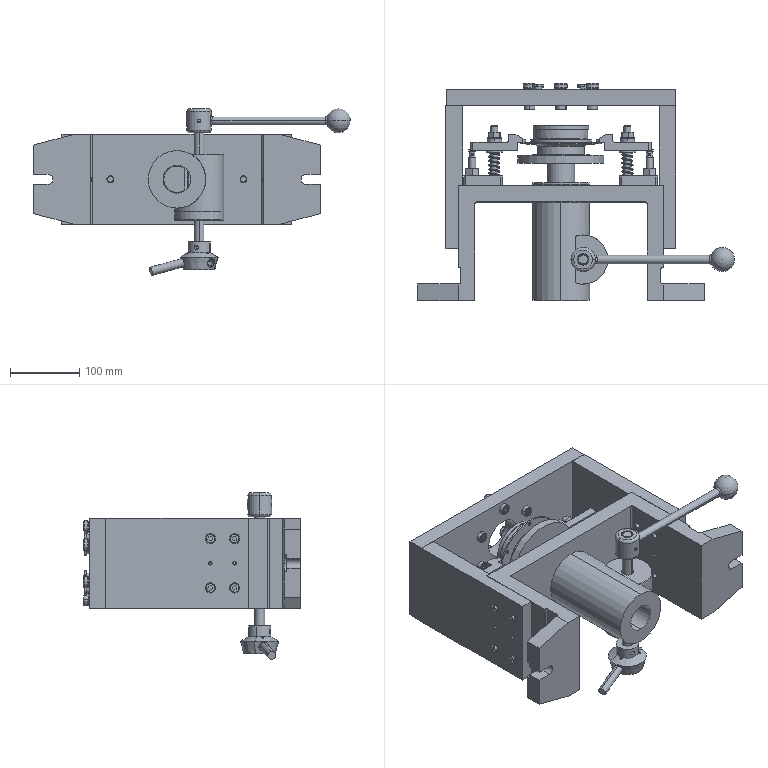Assembly | SolidWorks | mm | 72 component files | 73 solids | 1770 faces | box 457.51 x 313.05 x 240.63 mm | volume 5623344 mm3 | plane 629 | cylinder 586 | cone 407 | torus 132 | sphere 10 | spline 6 | commonest cylinder face diameters 15 x82 10 x68 5 x60 8 x58 6 x28 9 x24 9.5 x24 13 x24
Bill of materials:
CylindricalHelicalCompressionSpring | 2 |  | Helical coil of round wire with constant diameter and roughly uniform pitch, about six turns, with open cut ends.
CylindricalPin-UnhardenedSteelAndAusteniticStainlessSteel5_20 | 4 |  | Short solid cylindrical pin with a small chamfer at both ends. Its length is about four times its diameter.
CylindricalPin-UnhardenedSteelAndAusteniticStainlessSteel5_35 | 3 |  | Slender solid cylindrical pin with small chamfers at both ends. Its length is about seven times its diameter.
DrillJigBody | 1 |  | U-shaped channel bracket. Outward flanges at its base each have an open-ended slot. The side walls have small holes. A cylindrical boss with an axial through bore and a small radial cross hole sits inside the channel.
DrillTemplate | 1 |  | Flat rectangular plate with a large central through hole. Six smaller holes are spaced evenly around the central hole, and there are further holes near both short edges.
GB_T_70.1-2008[SocketHeadCapScrew_M4_20] | 3 |  | Solid of revolution with a short, larger-diameter cylindrical head and a smooth, plain cylindrical shank; the free end of the shank is chamfered. Looks like a headed screw blank or headed pin.
GB_T_70.1-2008[SocketHeadCapScrew_M8_30] | 12 |  | Socket-head-style fastener shape: a cylindrical head with a hexagonal recess in its end face, a smooth cylindrical shank, and a chamfered shank tip. Thread geometry is not modeled.
GB_T15389-1994ScrewM10_100 | 2 |  | Slender solid cylindrical pin. One end has a longer taper or chamfer than the other, which has a small chamfer.
GB_T6170-2000Type1HexNutA-gradeAndB-gradeM10 | 2 |  | Hexagonal nut-like body with a central round through bore. The axial length is short compared with the across-flats width, and the corners are chamfered.
GB_T6170-2015[Type1HexNutM12] | 2 |  | Hexagonal nut-like body with a central round through bore. Both ends have curved corner chamfers, and it is taller relative to its width than unnamed part.
GB_T95-2002[FlatWasherC-grade12] | 2 |  | Flat annular washer-like ring with a plain round central hole.
Handle | 1 |  | Lever or handle with a cylindrical hub at one end, a slender straight rod, and a spherical knob at the other end. The hub has an axial through bore and a small radial cross hole.
HandleRod10InMulti-HandleNut | 1 | Nickel | Solid stepped cylindrical shaft or pin: a long larger-diameter section with a shorter reduced-diameter section at one end.
Handwheel | 1 |  | Shaft carrying a toothed section like a spur gear next to a barrel-shaped (convex) section. There is a small cross hole near one end of the shaft.
JB_T8010.10-1999ElbowClampPlateTypeA12 | 2 | Nickel | Elongated prismatic block with chamfered corners in plan, a central oblong (stadium) through-slot, and a stepped, hook-like end profile in side view.
JB_T8013.1-1999LocatingBushingA18 | 6 | Nickel | Plain hollow cylindrical tube/sleeve with small chamfers at both ends.
Adjusting Support M16 | 2 | Nickel | Long cylindrical pin. At one end is a domed head with a short collar, then a reduced-diameter neck with a transverse through-hole, then a long main body ending in a chamfered tip.
JB_T8045.3-1999QuickChangeDrillBushing10_5_30 | 6 | Nickel | Headed cylindrical pin resembling a cap-screw form: chamfered cylindrical head, short reduced collar/undercut beneath it, plain shank with chamfered tip, and an axial bore; the head appears partially cut away.
JB_T8045.5-1999DrillBushingScrewM6 | 6 | Nickel | Stepped turned pin with a large disc-shaped head, an intermediate cylindrical step, a neck groove, and a chamfered small-diameter pin end; a small notch is cut into the head rim.
LocatingAxis | 1 |  | Pin with a thin large-diameter flat disc head and a cylindrical shank having a flat along part of its side and thread-like serrations near the free end.
LocatingPinAxis | 1 |  | Large chamfered disc with a small stepped hub on one face, comprising a thin flange ring and a short chamfered cylindrical stub.
Nut15InMulti-HandleNut | 1 | Nickel | Turned hub with a cylindrical boss on top of a frustoconical/flared base, a central through bore, radial holes in boss and base, and three axial holes in the base.
PressurePlateFixingSeat | 2 |  | Rectangular block with chamfered corners in plan and two round through holes along its long axis.
SealingCover | 1 |  | Flat circular flange/disc with a central through hole, an annular recess or counterbore on one face, and three small through holes evenly spaced near the perimeter.
SphericalWasherA21 | 2 | Nickel | Dished/conical washer with a convex curved face, flat opposite face, thin cylindrical outer rim, and central hole.
SphericalWasherB21 | 2 | Nickel | Plain flat annular ring/washer with rectangular cross-section.
SupportPlate | 2 |  | Rectangular plate with a thickness step across its width and a pattern of six through holes in two columns of three (four larger, two smaller in the middle row).
TurbineBearingHousing | 1 |  | Thin-walled, axisymmetric, open-ended tubular spigot with a thin flat annular flange. The flange has six evenly spaced through-holes on a bolt circle. On one side of the flange the sleeve steps out to a short collar of larger diameter, then into a main cylindrical section with a slightly raised lip at its far end. On the other side a short tapered shoulder leads to a plain cylindrical sleeve. There is a small oblong slot in the wall near the collar.
Mates:
1. coordinate | DrillJigBody-1 sketch point at (0, 0, 0) dir (1, 0, 0) | assembly sketch point at (0, 0, 0) dir (1, 0, 0)
2. concentric | DrillJigBody-1 face at (-147.862, 95, 35.5) dir (-1, 0, 0) r 4 | SupportPlate-1 face at (-165.862, 95, 35.5) dir (-1, 0, 0) r 7.5
3. concentric | DrillJigBody-1 face at (-147.862, 95, -35.5) dir (-1, 0, 0) r 4 | SupportPlate-1 face at (-165.862, 95, -35.5) dir (-1, 0, 0) r 4.5
4. coincident | DrillJigBody-1 face at (-147.862, 47.316, 65) dir (-1, 0, 0) | SupportPlate-1 face at (-147.862, 75, -99) dir (1, 0, 0)
5. concentric | DrillJigBody-1 face at (0, -23.394, 0) dir (0, 1, 0) r 20 | assembly face at (0, 30.606, 0) dir (0, 1, 0) r 23.5
6. parallel | assembly plane at (0, 197.606, 0) dir (-1, 0, 0) | assembly plane at (0, 0, 0) dir (1, 0, 0)
7. distance | assembly face at (0, 185.606, 0) dir (0, -1, 0) | DrillJigBody-1 face at (0, 169.606, 0) dir (0, 1, 0)
8. concentric | TurbineBearingHousing-1 face at (0, 209.806, 0) dir (0, -1, 0) r 33.75 | DrillJigBody-1 face at (0, -0.05241, 0) dir (0, 1, 0) r 41.5
9. distance | TurbineBearingHousing-1 face at (-57.998, 227.606, -0.4799) dir (0, 1, 0) | DrillJigBody-1 face at (-147.862, 165.606, 65) dir (0, 1, 0)
10. distance | assembly face at (29.76, 42.6, 59) dir (0, 0, 1) | DrillJigBody-1 face at (32, 58.948, 47) dir (0, 0, 1)
11. concentric | DrillJigBody-1 face at (32, 58.948, 81.865) dir (0, 0, 1) r 17.918 | assembly face at (32, 58.948, 112) dir (0, 0, -1) r 7.5
12. concentric | assembly face at (32, 58.948, 112) dir (0, 0, -1) r 7.5 | assembly face at (32, 58.948, 59) dir (0, 0, 1) r 7.5
13. concentric | DrillJigBody-1 face at (32, 29.448, 47) dir (0, 0, 1) r 1.65 | assembly face at (32, 29.448, 59) dir (0, 0, 1) r 2.25
14. coincident | DrillJigBody-1 face at (32, 58.948, 47) dir (0, 0, 1) | assembly face at (32, 58.948, 47) dir (0, 0, -1)
15. concentric | assembly face at (32, 58.948, 112) dir (0, 0, -1) r 7.5 | assembly face at (32, 58.948, 130.416) dir (0, 0, 1) r 9
16. distance | assembly face at (32, 58.948, 112) dir (0, 0, 1) | assembly face at (32, 58.948, 130.416) dir (0, 0, 1)
17. concentric | assembly face at (55.39, 68.739, 120.416) dir (0.891, 0.373, 0.2588) r 5 | assembly face at (53.608, 67.993, 119.898) dir (-0.891, -0.373, -0.2588) r 5
18. coincident | assembly face at (54.382, 64.065, 122.893) dir (0.891, 0.373, 0.2588) | assembly face at (53.608, 67.993, 119.898) dir (-0.891, -0.373, -0.2588)
19. concentric | SupportPlate-1 face at (-153.5, 281, 27.5) dir (0, 1, 0) r 4 | DrillTemplate-1 face at (-153.5, 305, 27.5) dir (0, 1, 0) r 7.5
20. concentric | SupportPlate-1 face at (-153.5, 281, -27.5) dir (0, 1, 0) r 4 | DrillTemplate-1 face at (-153.5, 305, -27.5) dir (0, 1, 0) r 7.5
21. coincident | SupportPlate-1 face at (-141.862, 281, -65) dir (0, 1, 0) | DrillTemplate-1 face at (0, 281, 0) dir (0, -1, 0)
22. concentric | DrillTemplate-1 face at (0, 305, 52.5) dir (0, 1, 0) r 7.5 | JB_T8013.1-1999LocatingBushingA18-1 face at (0, 275, 52.5) dir (0, 1, 0) r 7.5
23. coincident | DrillTemplate-1 face at (0, 305, 0) dir (0, 1, 0) | JB_T8013.1-1999LocatingBushingA18-1 face at (0, 305, 52.5) dir (0, 1, 0)
24. concentric | JB_T8013.1-1999LocatingBushingA18-1 face at (0, 275, 52.5) dir (0, 1, 0) r 5 | JB_T8045.3-1999QuickChangeDrillBushing10_5_30-1 face at (0, 415.352, 52.5) dir (0, 1, 0) r 5
25. coincident | JB_T8013.1-1999LocatingBushingA18-1 face at (0, 305, 52.5) dir (0, 1, 0) | JB_T8045.3-1999QuickChangeDrillBushing10_5_30-1 face at (0, 305, 45) dir (0, -1, 0)
26. parallel | DrillTemplate-1 face at (-165.5, 281, 65) dir (0, 0, 1) | JB_T8045.3-1999QuickChangeDrillBushing10_5_30-1 face at (68.423, 408, 47) dir (0, 0, -1)
27. concentric | DrillTemplate-1 face at (0, 305, 37.5) dir (0, 1, 0) r 3 | JB_T8045.5-1999DrillBushingScrewM6-1 face at (0, 294, 37.5) dir (0, 1, 0) r 3
28. coincident | JB_T8045.3-1999QuickChangeDrillBushing10_5_30-1 face at (68.423, 308, 47) dir (0, 1, 0) | JB_T8045.5-1999DrillBushingScrewM6-1 face at (0, 308, 37.5) dir (0, -1, 0)
29. angle | JB_T8045.5-1999DrillBushingScrewM6-1 face at (17.932, 310, 56.492) dir (0.7071, 0, -0.7071) | JB_T8045.3-1999QuickChangeDrillBushing10_5_30-1 face at (68.423, 408, 47) dir (0, 0, -1)
30. parallel | TurbineBearingHousing-1 face at (-0.4344, 227.606, 52.498) dir (0, 1, 0) r 2.75 | JB_T8045.3-1999QuickChangeDrillBushing10_5_30-1 face at (0, 415.352, 52.5) dir (0, 1, 0) r 2.5
31. concentric | DrillJigBody-1 face at (96, 165.606, 0) dir (0, 1, 0) r 5 | JB_T8010.10-1999ElbowClampPlateTypeA12-1 face at (96, 223.606, 0) dir (0, -1, 0) r 7.5
32. coincident | TurbineBearingHousing-1 face at (-57.998, 227.606, -0.4799) dir (0, 1, 0) | JB_T8010.10-1999ElbowClampPlateTypeA12-1 face at (51, 227.606, 16) dir (0, -1, 0)
33. parallel | SupportPlate-2 face at (141.862, 75, 65) dir (0, 0, 1) | JB_T8010.10-1999ElbowClampPlateTypeA12-1 face at (51, 223.606, 16) dir (0, 0, 1)
34. concentric | DrillJigBody-1 face at (128, 165.606, 0) dir (0, 1, 0) r 5 | JB_T8026.4-1999AdjustingSupportM10_40-1 face at (128, 262.155, 0) dir (0, 1, 0) r 5
35. tangent | JB_T8010.10-1999ElbowClampPlateTypeA12-1 face at (51, 218.606, 0) dir (0, -1, 0) | JB_T8026.4-1999AdjustingSupportM10_40-1 face at (128, 208.606, 0) dir (1, 0, 0) r 10
36. concentric | DrillJigBody-1 face at (96, 165.606, 0) dir (0, 1, 0) r 5 | GB_T15389-1994ScrewM10_100-1 face at (96, 171.901, 0) dir (0, 1, 0) r 5
37. distance | GB_T15389-1994ScrewM10_100-1 face at (96, 251.901, 0) dir (0, 1, 0) | GB_T6170-2000Type1HexNutA-gradeAndB-gradeM10-3 face at (87.661, 242.901, -3.066) dir (0, 1, 0)
38. concentric | GB_T15389-1994ScrewM10_100-1 face at (96, 171.901, 0) dir (0, 1, 0) r 5 | assembly face at (96, 174.006, 0) dir (0, -1, 0) r 5
39. coincident | DrillJigBody-1 face at (-147.862, 165.606, 65) dir (0, 1, 0) | assembly face at (103.712, 165.606, -4.412) dir (0, -1, 0)
40. concentric | JB_T8026.4-1999AdjustingSupportM10_40-1 face at (128, 262.155, 0) dir (0, 1, 0) r 5 | assembly face at (128, 165.606, 0) dir (0, 1, 0) r 5
41. coincident | DrillJigBody-1 face at (-147.862, 165.606, 65) dir (0, 1, 0) | assembly face at (123.957, 165.606, -7.912) dir (0, -1, 0)
42. concentric | GB_T15389-1994ScrewM10_100-1 face at (96, 171.901, 0) dir (0, 1, 0) r 5 | SphericalWasherB21-1 face at (96, 238.624, 0) dir (0, 1, 0) r 5.75
43. coincident | JB_T8010.10-1999ElbowClampPlateTypeA12-1 face at (131, 228.606, -16) dir (0, 1, 0) | SphericalWasherB21-1 face at (101.75, 228.606, 0) dir (0, -1, 0)
44. concentric | GB_T15389-1994ScrewM10_100-1 face at (96, 171.901, 0) dir (0, 1, 0) r 5 | SphericalWasherA21-1 face at (96, 230.466, 0) dir (0, -1, 0) r 5.25
45. tangent | SphericalWasherA21-1 face at (96, 244.553, 0) dir (1, 0, 0) r 15 | SphericalWasherB21-1 face at (96, 233.006, 0) dir (0, -1, 0) r 1047.198
46. concentric | GB_T15389-1994ScrewM10_100-1 face at (96, 171.901, 0) dir (0, 1, 0) r 5 | GB_T6170-2000Type1HexNutA-gradeAndB-gradeM10-3 face at (96, 234.501, 0) dir (0, 1, 0) r 5
47. coincident | SphericalWasherA21-1 face at (97.393, 234.501, -5.062) dir (0, 1, 0) | GB_T6170-2000Type1HexNutA-gradeAndB-gradeM10-3 face at (87.661, 234.501, -3.066) dir (0, -1, 0)
48. concentric | assembly face at (32, 58.948, -20) dir (0, 0, -1) r 7.5 | Handle-1 face at (32, 58.948, 102) dir (0, 0, -1) r 17.5
49. coincident | Handle-1 face at (32, 58.948, 102) dir (0, 0, 1) | Handwheel-2 face at (32, 58.948, 102) dir (0, 0, 1)
50. parallel | DrillTemplate-1 face at (0, 305, 0) dir (0, 1, 0) | Handle-1 plane at (32, 58.948, 84.5) dir (0, -1, 0)
51. concentric | Nut15InMulti-HandleNut-3 face at (32, 58.948, -130.416) dir (0, 0, -1) r 9 | Handwheel-2 face at (32, 58.948, -112) dir (0, 0, 1) r 7.5
52. concentric | SealingCover-2 face at (32, 58.948, -59) dir (0, 0, -1) r 7.5 | Handwheel-2 face at (32, 58.948, -112) dir (0, 0, 1) r 7.5
53. distance | Handwheel-2 face at (32, 58.948, -112) dir (0, 0, -1) | Nut15InMulti-HandleNut-3 face at (32, 58.948, -130.416) dir (0, 0, -1)
54. coincident | HandleRod10InMulti-HandleNut-2 face at (9.315, 53.107, -119.898) dir (0.9354, 0.2408, 0.2588) | Nut15InMulti-HandleNut-3 face at (11.071, 49.509, -122.893) dir (-0.9354, -0.2408, -0.2588)
55. concentric | HandleRod10InMulti-HandleNut-2 face at (9.315, 53.107, -119.898) dir (0.9354, 0.2408, 0.2588) r 5 | Nut15InMulti-HandleNut-3 face at (7.444, 52.625, -120.416) dir (-0.9354, -0.2408, -0.2588) r 5
56. concentric | DrillJigBody-1 face at (32, 58.948, 36) dir (0, 0, -1) r 35.5 | Handwheel-2 face at (32, 58.948, -112) dir (0, 0, 1) r 7.5
57. coincident | DrillJigBody-1 face at (32, 58.948, -47) dir (0, 0, -1) | SealingCover-2 face at (32, 58.948, -47) dir (0, 0, 1)
58. concentric | DrillJigBody-1 face at (32, 29.448, -47) dir (0, 0, -1) r 2 | SealingCover-2 face at (32, 29.448, -59) dir (0, 0, -1) r 4
59. distance | Handwheel-2 face at (32, 58.948, 102) dir (0, 0, 1) | DrillJigBody-1 face at (121.838, 139.582, 65) dir (0, 0, 1)
60. concentric | Handle-1 face at (32, 58.948, 102) dir (0, 0, -1) r 17.5 | Handwheel-2 face at (32, 58.948, 20) dir (0, 0, 1) r 7.5
61. concentric | Handle-1 face at (32, 76.448, 84.5) dir (0, -1, 0) r 2.5 | Handwheel-2 face at (32, 39.338, 84.5) dir (0, 1, 0) r 2.5
62. concentric | Handle-1 face at (32, 76.448, 84.5) dir (0, -1, 0) r 2.5 | CylindricalPin-UnhardenedSteelAndAusteniticStainlessSteel5_35-1 face at (32, 41.448, 84.5) dir (0, 1, 0) r 2.5
63. tangent | Handle-1 face at (32, 58.948, 102) dir (0, 0, -1) r 17.5 | CylindricalPin-UnhardenedSteelAndAusteniticStainlessSteel5_35-1 face at (32, 76.448, 84.5) dir (0, 1, 0)
64. concentric | SupportPlate-2 face at (165.862, 130, 0) dir (1, 0, 0) r 2.5 | CylindricalPin-UnhardenedSteelAndAusteniticStainlessSteel5_20-1 face at (159.862, 130, 0) dir (-1, 0, 0) r 2.5
65. distance | CylindricalPin-UnhardenedSteelAndAusteniticStainlessSteel5_20-1 face at (159.862, 130, 0) dir (1, 0, 0) | SupportPlate-2 face at (165.862, 75, 0) dir (1, 0, 0)
66. concentric | SupportPlate-2 face at (165.862, 95, 0) dir (1, 0, 0) r 2.5 | CylindricalPin-UnhardenedSteelAndAusteniticStainlessSteel5_20-2 face at (159.862, 95, 0) dir (-1, 0, 0) r 2.5
67. distance | CylindricalPin-UnhardenedSteelAndAusteniticStainlessSteel5_20-2 face at (159.862, 95, 0) dir (1, 0, 0) | SupportPlate-2 face at (165.862, 75, 0) dir (1, 0, 0)
68. coincident | SupportPlate-2 face at (156.862, 130, 31) dir (1, 0, 0) | GB_T_70.1-2008[SocketHeadCapScrew_M8_30]-1 face at (156.862, 127.518, 41.507) dir (-1, 0, 0)
69. concentric | SupportPlate-2 face at (165.862, 130, 35.5) dir (1, 0, 0) r 7.5 | GB_T_70.1-2008[SocketHeadCapScrew_M8_30]-1 face at (164.862, 130, 35.5) dir (-1, 0, 0) r 4
70. coincident | DrillJigBody-1 face at (-147.862, 165.606, 65) dir (0, 1, 0) | PressurePlateFixingSeat-1 face at (112, 165.606, 0) dir (0, -1, 0)
71. concentric | GB_T15389-1994ScrewM10_100-1 face at (96, 171.901, 0) dir (0, 1, 0) r 5 | PressurePlateFixingSeat-1 face at (96, 179.606, 0) dir (0, 1, 0) r 5.1
72. parallel | SupportPlate-2 face at (141.862, 75, 0) dir (-1, 0, 0) | PressurePlateFixingSeat-1 face at (84, 179.606, 15) dir (-1, 0, 0)
73. concentric | JB_T8026.4-1999AdjustingSupportM10_40-1 face at (128, 262.155, 0) dir (0, 1, 0) r 5 | GB_T6170-2015[Type1HexNutM12]-1 face at (128, 190.406, 0) dir (0, -1, 0) r 5.053
74. coincident | PressurePlateFixingSeat-1 face at (112, 179.606, 0) dir (0, 1, 0) | GB_T6170-2015[Type1HexNutM12]-1 face at (128, 179.606, 10.392) dir (0, -1, 0)
75. concentric | GB_T15389-1994ScrewM10_100-1 face at (96, 171.901, 0) dir (0, 1, 0) r 5 | GB_T95-2002[FlatWasherC-grade12]-1 face at (96, 205.461, 0) dir (0, -1, 0) r 12
76. coincident | JB_T8010.10-1999ElbowClampPlateTypeA12-1 face at (51, 216.606, 0) dir (0, -1, 0) | GB_T95-2002[FlatWasherC-grade12]-1 face at (89.25, 216.606, 0) dir (0, 1, 0)
77. concentric | GB_T15389-1994ScrewM10_100-1 face at (96, 171.901, 0) dir (0, 1, 0) r 5 | CylindricalHelicalCompressionSpring-1 axis at (96, 216.356, 0) dir (0, -1, 0)
78. coincident | GB_T95-2002[FlatWasherC-grade12]-1 face at (89.25, 214.106, 0) dir (0, -1, 0) | CylindricalHelicalCompressionSpring-1 face at (86.712, 214.106, -8) dir (0, 1, 0)
79. concentric | DrillTemplate-1 face at (-153.5, 305, -48) dir (0, 1, 0) r 2.5 | CylindricalPin-UnhardenedSteelAndAusteniticStainlessSteel5_35-2 face at (-153.5, 305, -48) dir (0, -1, 0) r 2.5
80. coincident | DrillTemplate-1 face at (0, 305, 0) dir (0, 1, 0) | CylindricalPin-UnhardenedSteelAndAusteniticStainlessSteel5_35-2 face at (-153.5, 305, -48) dir (0, 1, 0)
81. concentric | DrillTemplate-1 face at (-153.5, 305, 48) dir (0, 1, 0) r 2.5 | CylindricalPin-UnhardenedSteelAndAusteniticStainlessSteel5_35-3 face at (-153.5, 305, 48) dir (0, -1, 0) r 2.5
82. coincident | DrillTemplate-1 face at (0, 305, 0) dir (0, 1, 0) | CylindricalPin-UnhardenedSteelAndAusteniticStainlessSteel5_35-3 face at (-153.5, 305, 48) dir (0, 1, 0)
83. coincident | DrillTemplate-1 face at (-149, 296, 27.5) dir (0, 1, 0) | GB_T_70.1-2008[SocketHeadCapScrew_M8_30]-9 face at (-147, 296, 27.5) dir (0, -1, 0)
84. concentric | DrillTemplate-1 face at (-153.5, 305, 27.5) dir (0, 1, 0) r 7.5 | GB_T_70.1-2008[SocketHeadCapScrew_M8_30]-9 face at (-153.5, 304, 27.5) dir (0, -1, 0) r 6.5
85. coincident | DrillTemplate-1 face at (-149, 296, -27.5) dir (0, 1, 0) | GB_T_70.1-2008[SocketHeadCapScrew_M8_30]-10 face at (-147.116, 296, -28.725) dir (0, -1, 0)
86. concentric | DrillTemplate-1 face at (-153.5, 305, -27.5) dir (0, 1, 0) r 7.5 | GB_T_70.1-2008[SocketHeadCapScrew_M8_30]-10 face at (-153.5, 304, -27.5) dir (0, -1, 0) r 6.5
87. coincident | DrillTemplate-1 face at (158, 296, -27.5) dir (0, 1, 0) | GB_T_70.1-2008[SocketHeadCapScrew_M8_30]-12 face at (159.469, 296, -30.072) dir (0, -1, 0)
88. concentric | DrillTemplate-1 face at (153.5, 305, -27.5) dir (0, 1, 0) r 7.5 | GB_T_70.1-2008[SocketHeadCapScrew_M8_30]-12 face at (153.5, 304, -27.5) dir (0, -1, 0) r 6.5
89. coincident | DrillTemplate-1 face at (158, 296, 27.5) dir (0, 1, 0) | GB_T_70.1-2008[SocketHeadCapScrew_M8_30]-14 face at (158.7, 296, 23.6) dir (0, -1, 0)
90. concentric | DrillTemplate-1 face at (153.5, 305, 27.5) dir (0, 1, 0) r 7.5 | GB_T_70.1-2008[SocketHeadCapScrew_M8_30]-14 face at (153.5, 304, 27.5) dir (0, -1, 0) r 6.5
91. parallel | SupportPlate-1 face at (-165.862, 75, 0) dir (-1, 0, 0) | LocatingAxis-2 face at (15, 42.806, 62) dir (1, 0, 0)
92. coincident | TurbineBearingHousing-1 face at (-31.499, 209.806, -0.2606) dir (0, -1, 0) | LocatingAxis-2 face at (0, 209.806, 0) dir (0, 1, 0)
93. concentric | TurbineBearingHousing-1 face at (0, 209.806, 0) dir (0, -1, 0) r 31.5 | LocatingAxis-2 face at (0, 209.806, 0) dir (0, 1, 0) r 20
94. concentric | LocatingAxis-2 face at (0, 209.806, 0) dir (0, 1, 0) r 62 | LocatingPinAxis-1 face at (0, 191.806, 0) dir (0, -1, 0) r 31.5
95. coincident | LocatingAxis-2 face at (0, 209.806, 0) dir (0, 1, 0) | LocatingPinAxis-1 face at (10.916, 209.806, -6.091) dir (0, -1, 0)
96. coincident | SealingCover-2 face at (55.298, 73.698, -54.4) dir (0, 0, -1) | GB_T_70.1-2008[SocketHeadCapScrew_M4_20]-1 face at (57.548, 77.198, -54.4) dir (0, 0, 1)
97. concentric | SealingCover-2 face at (57.548, 73.698, -59) dir (0, 0, -1) r 4 | GB_T_70.1-2008[SocketHeadCapScrew_M4_20]-1 face at (57.548, 73.698, -58.4) dir (0, 0, 1) r 2